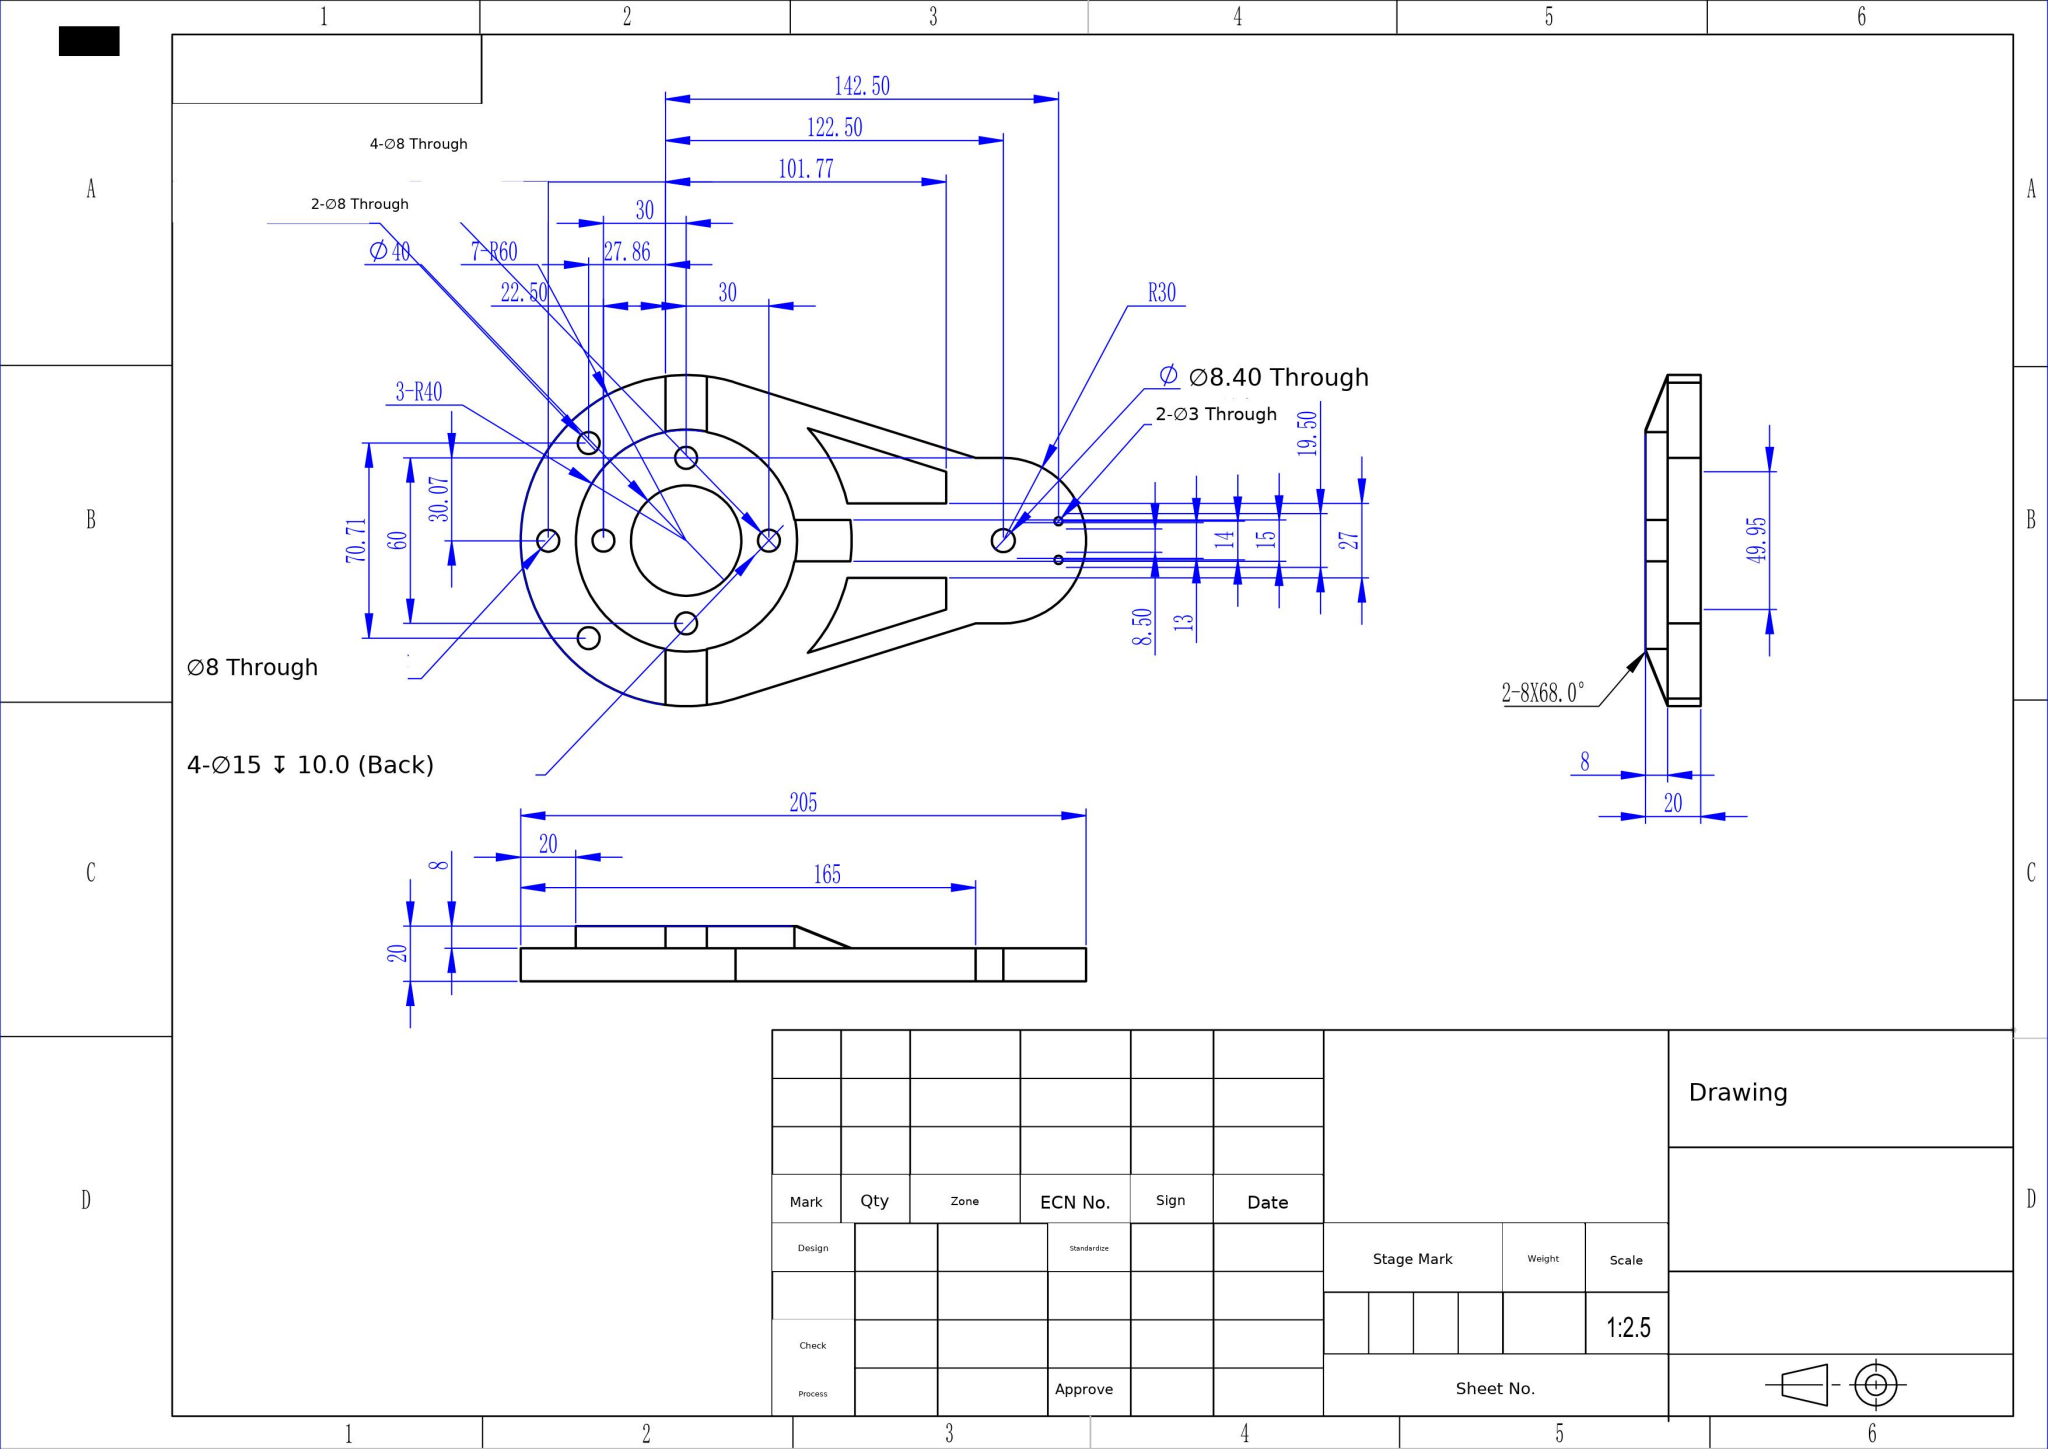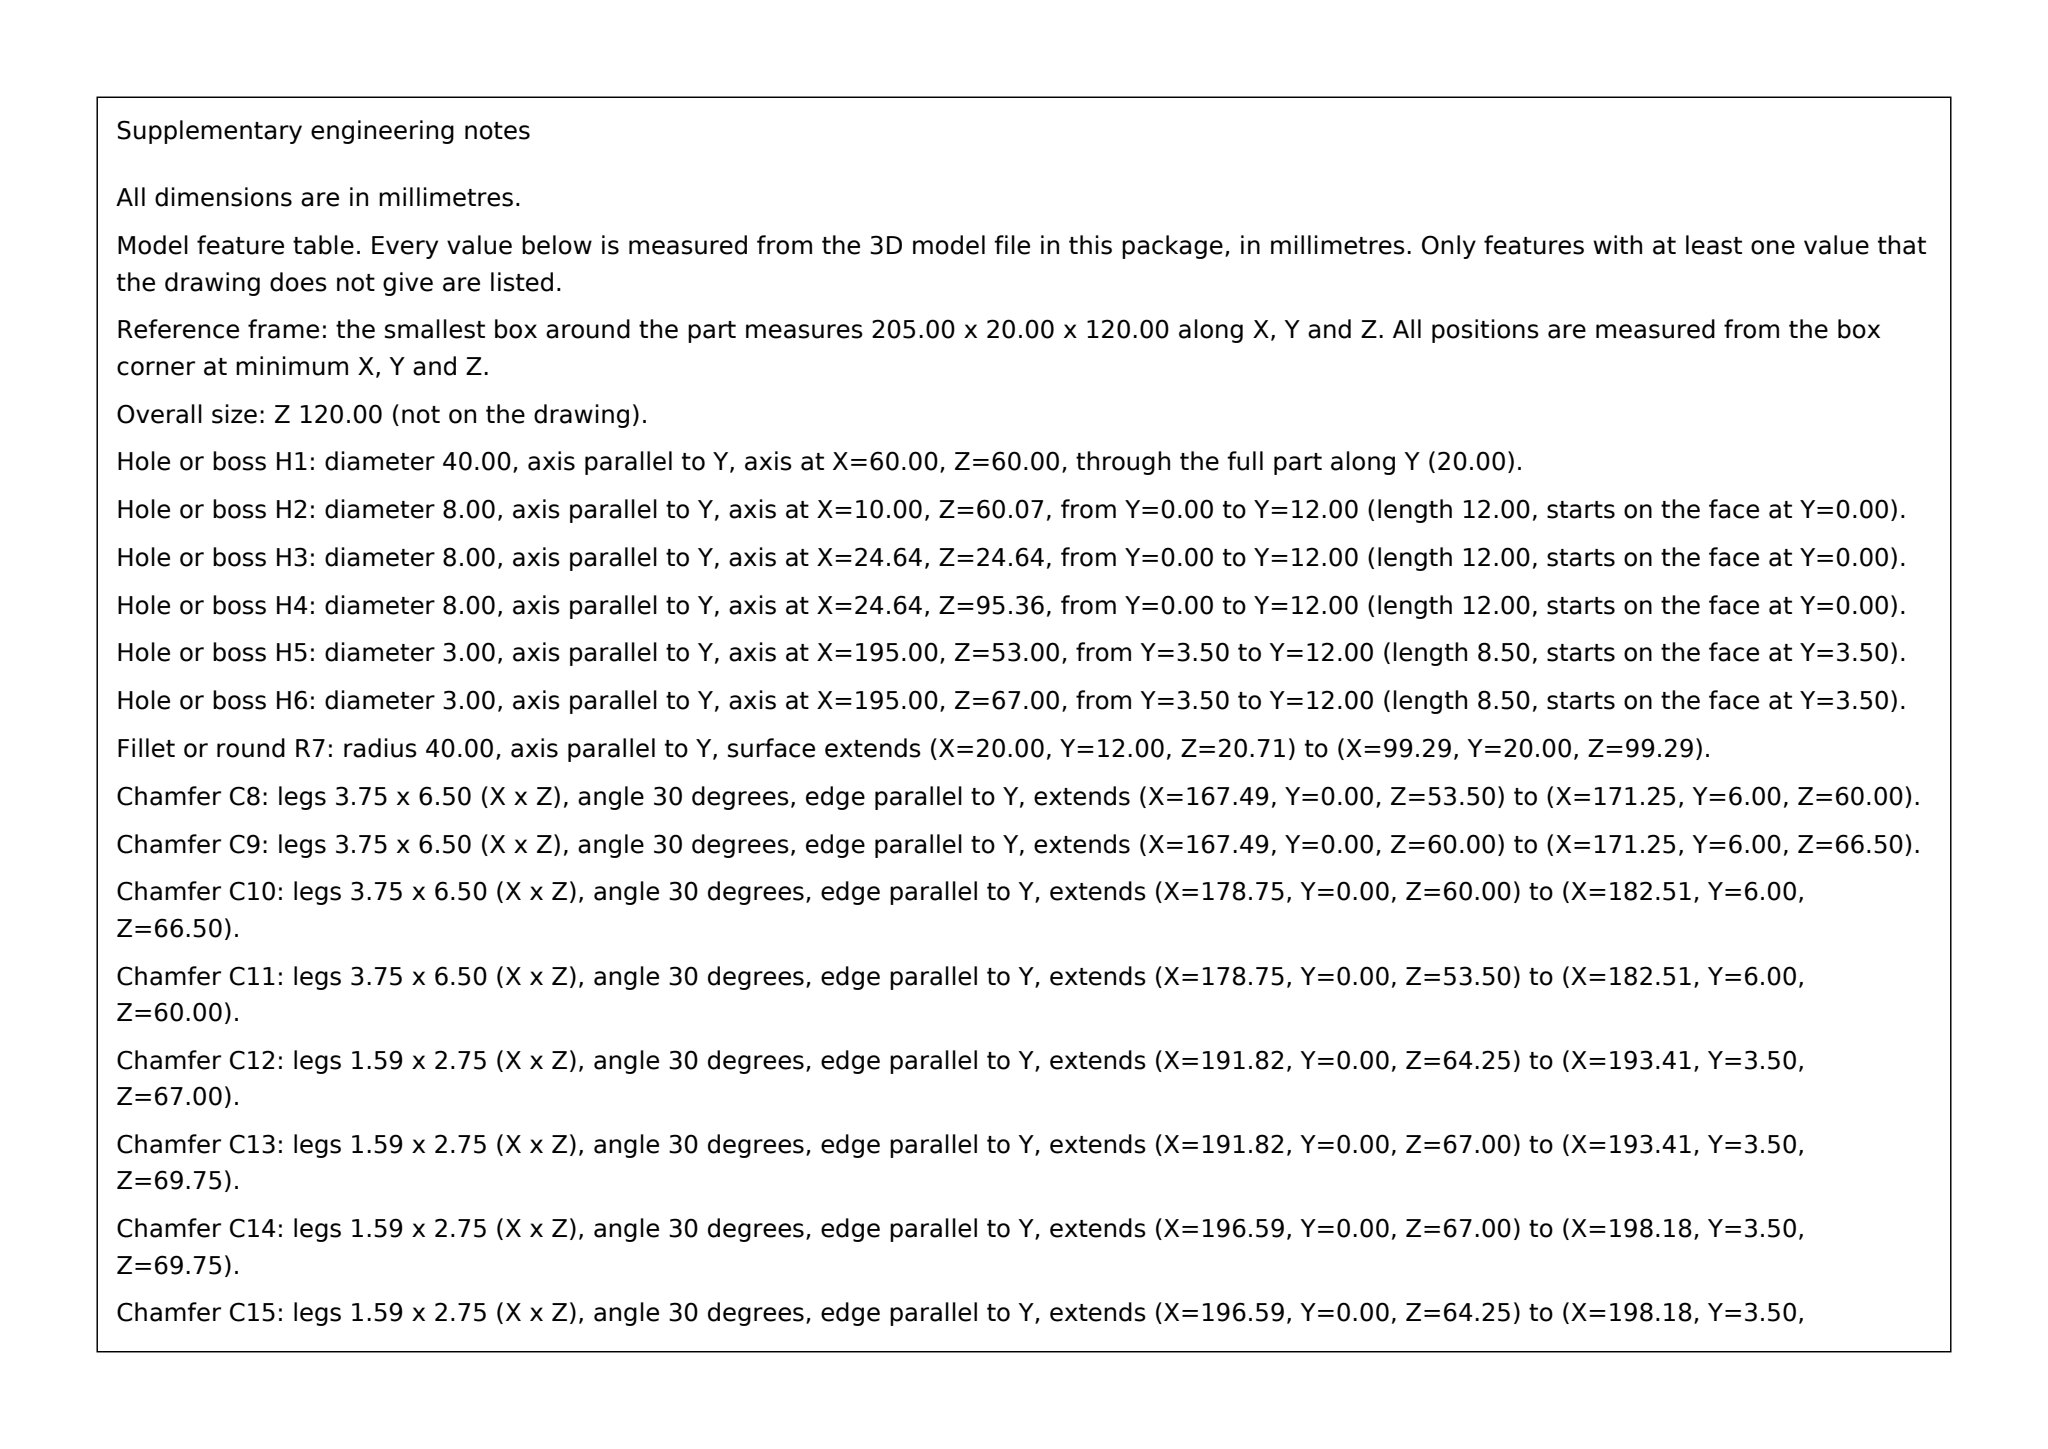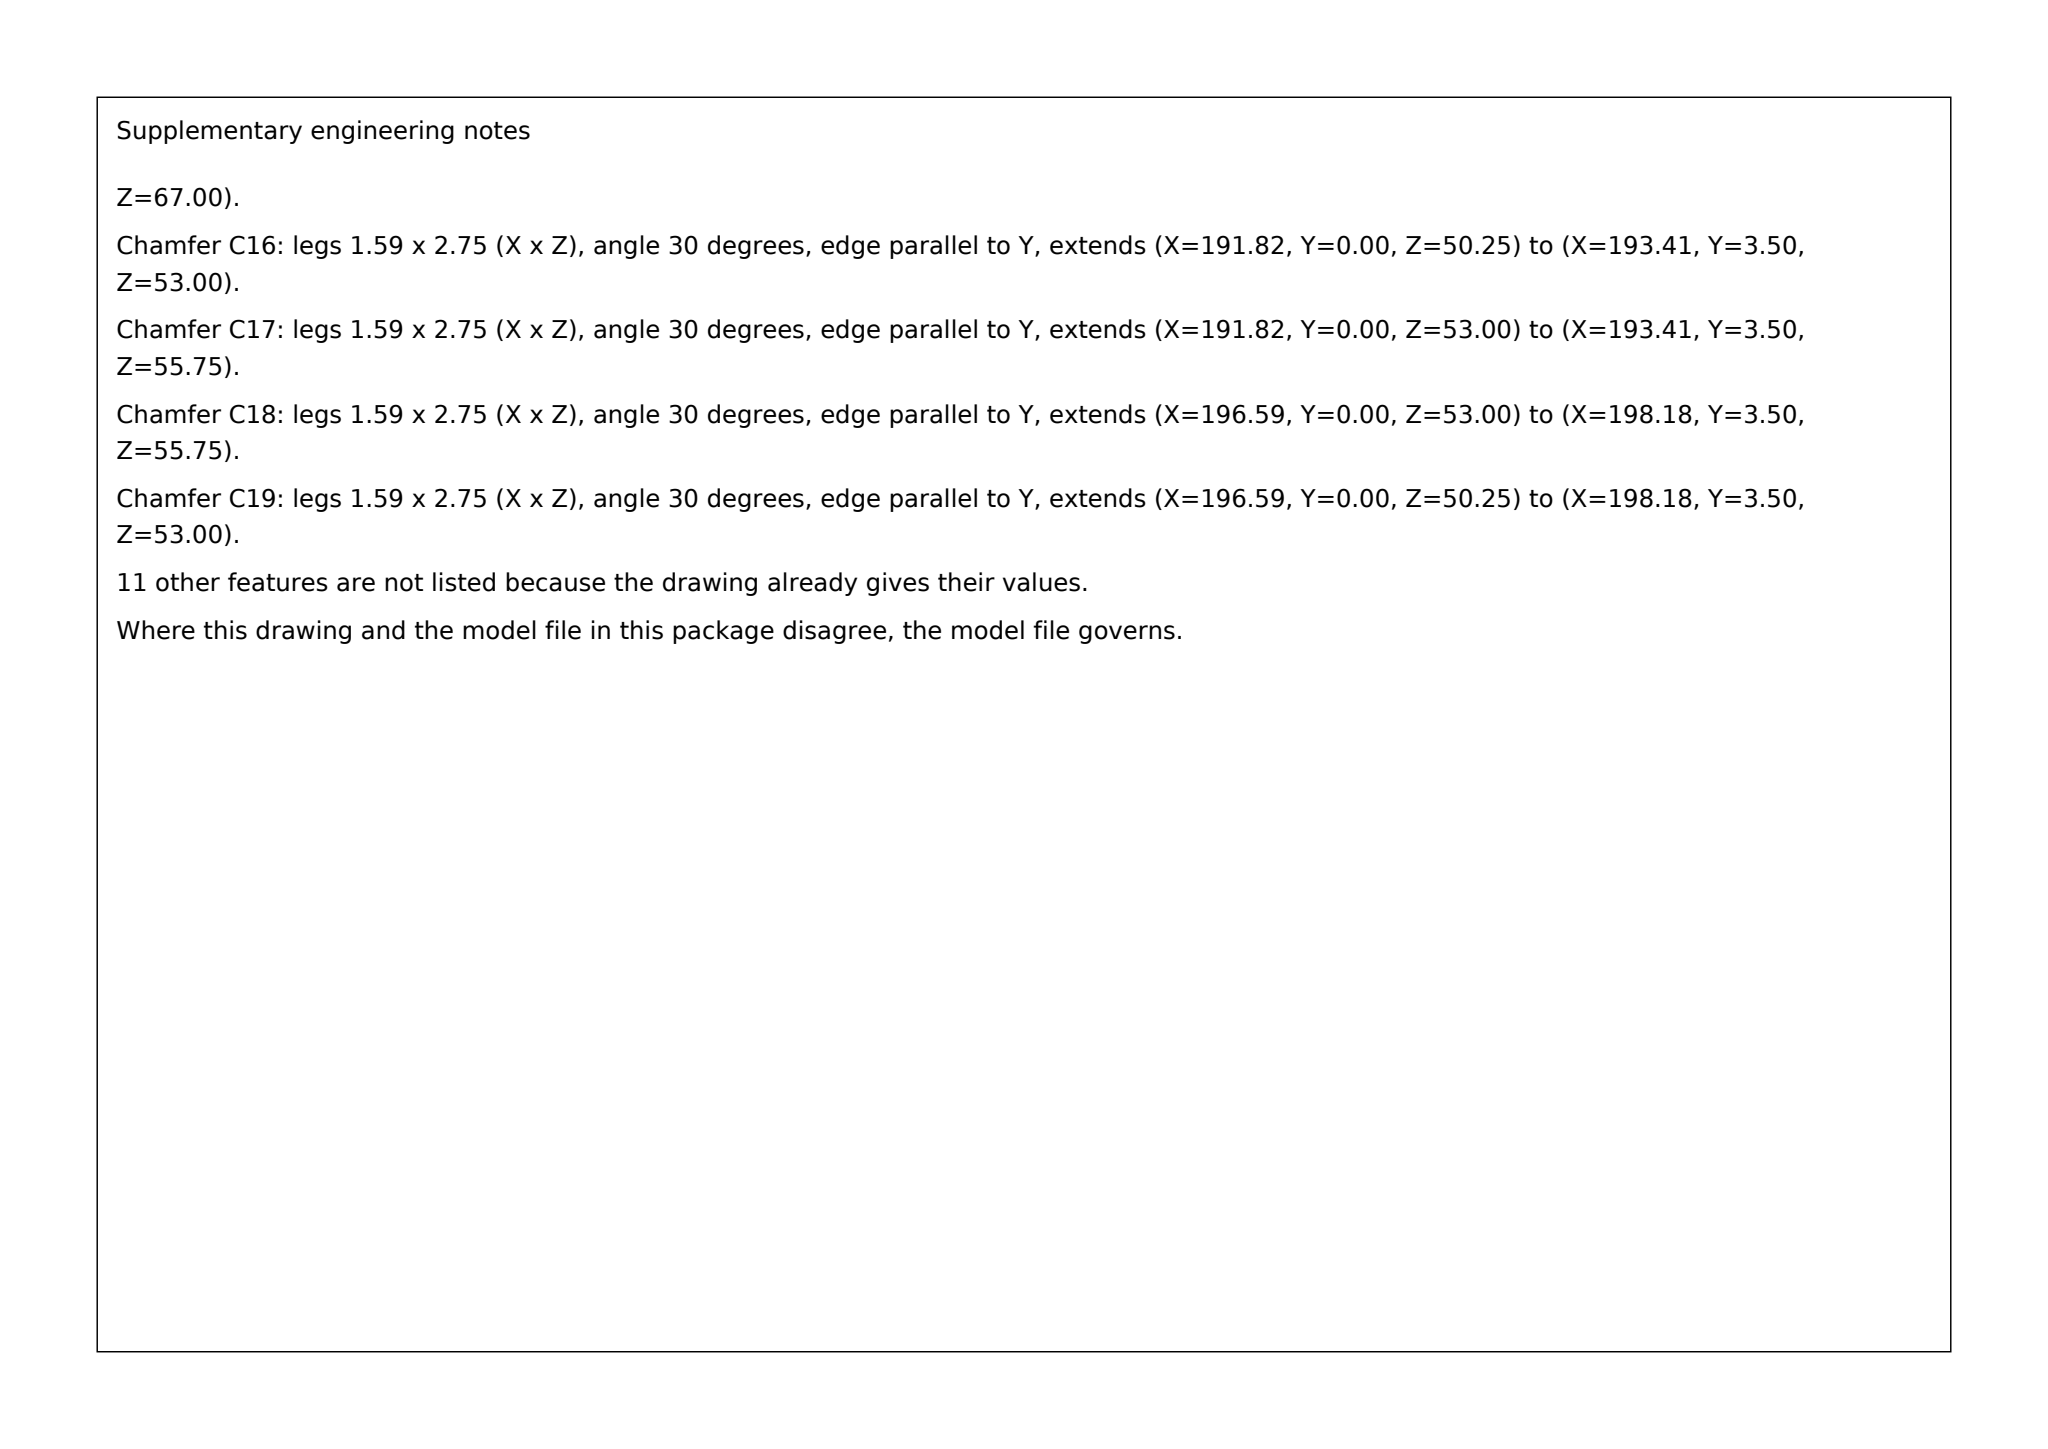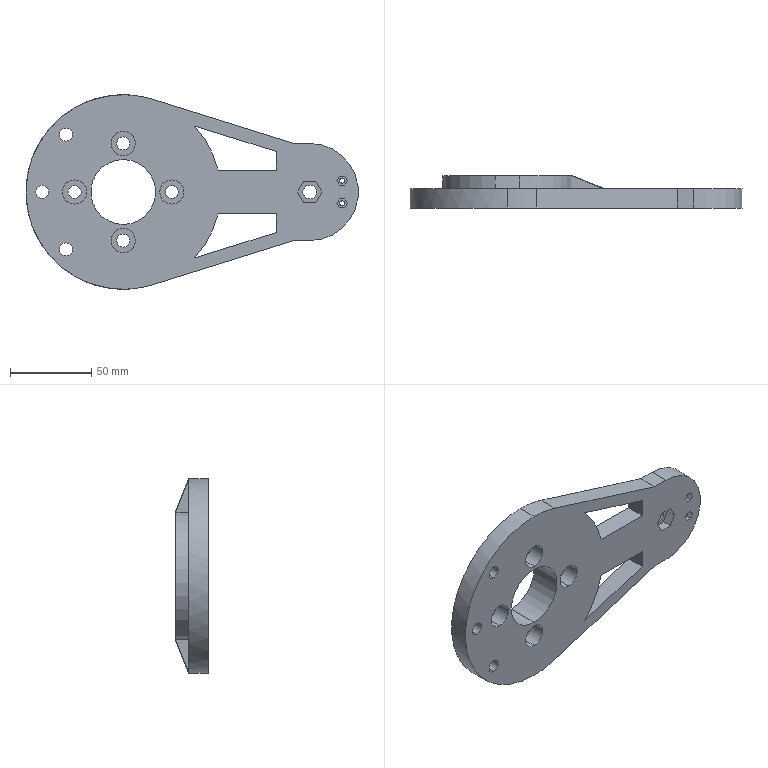Part | SolidWorks | mm | 1 solid | 88 faces | box 205 x 20 x 120 mm | volume 197352 mm3 | plane 45 | cylinder 39 | cone 4 | commonest cylinder face diameters 8 x14 15 x8 120 x5 3 x4 80 x3 8.4 x2 40 x2 60 x1